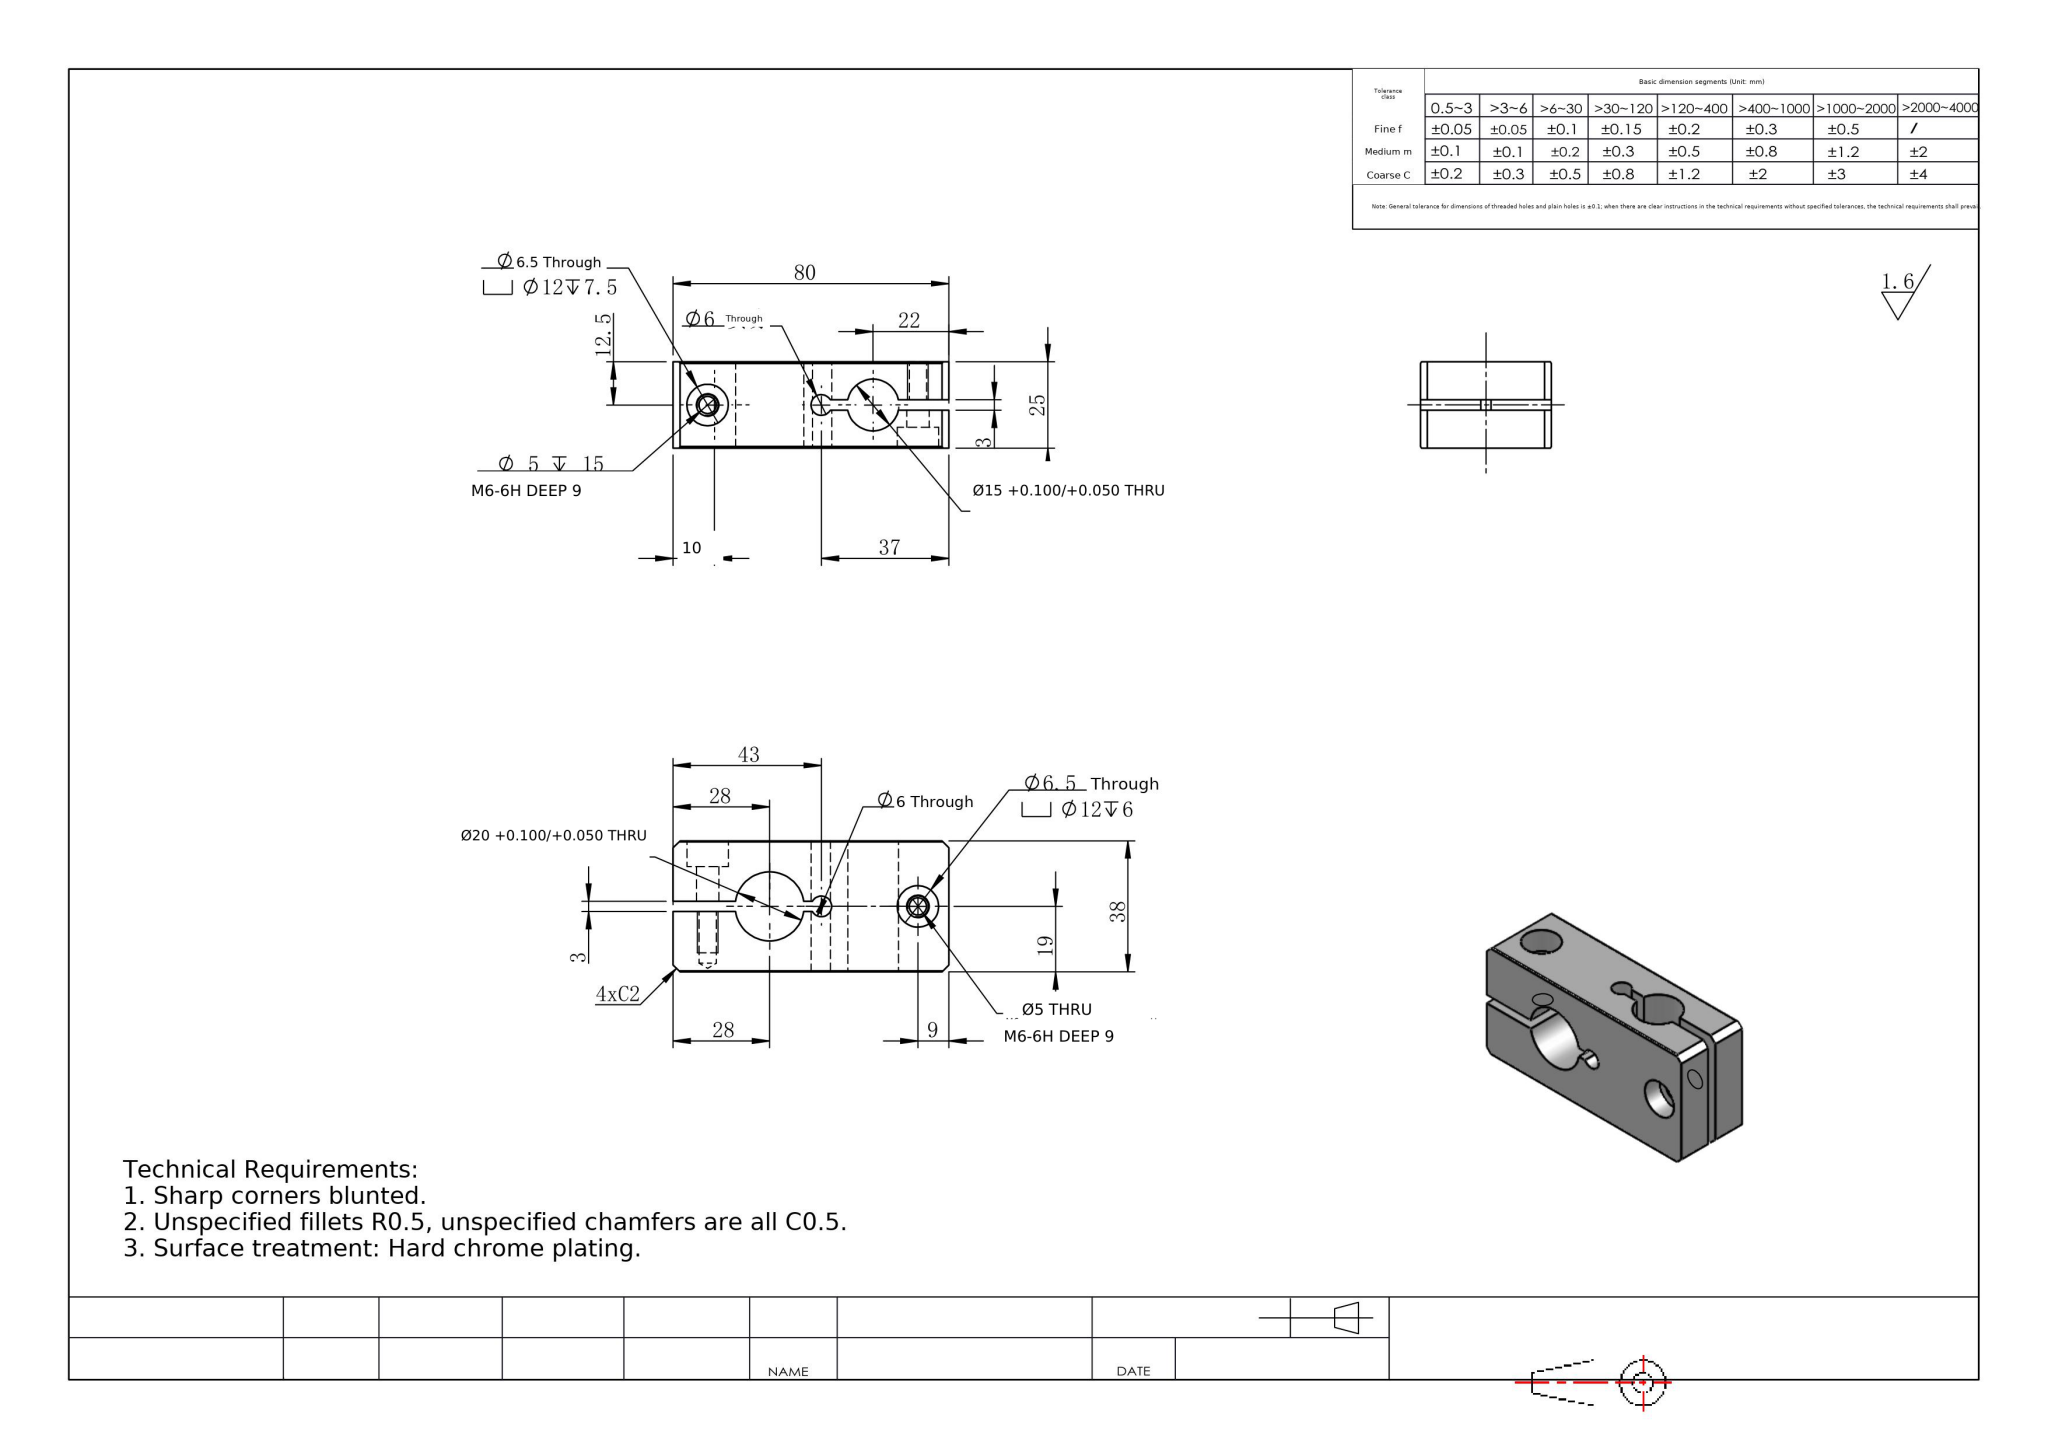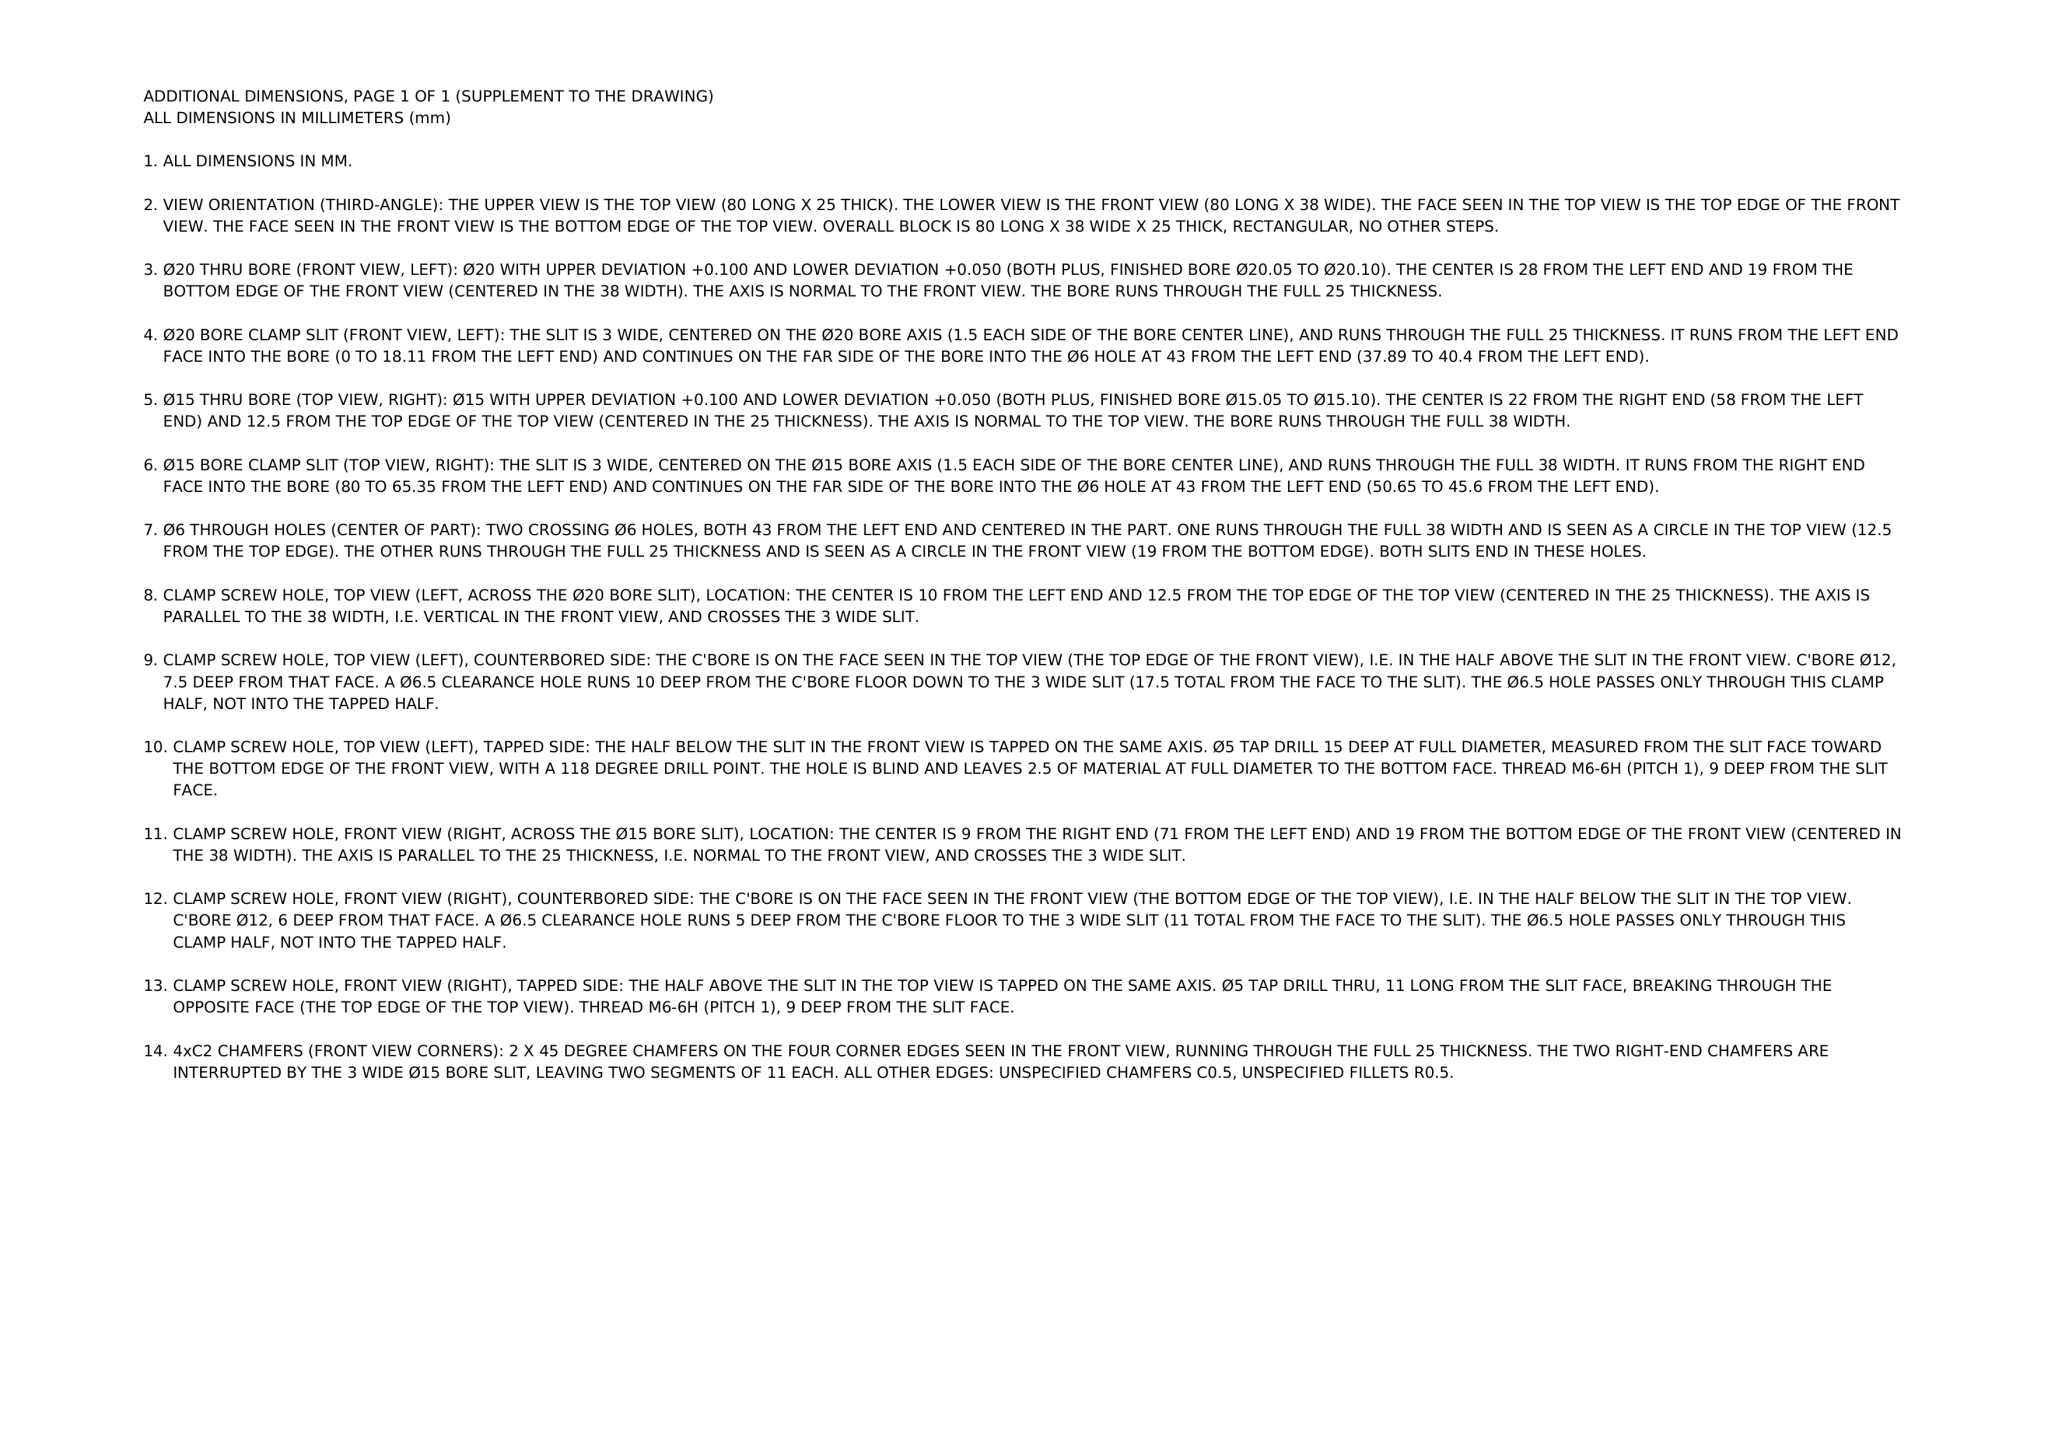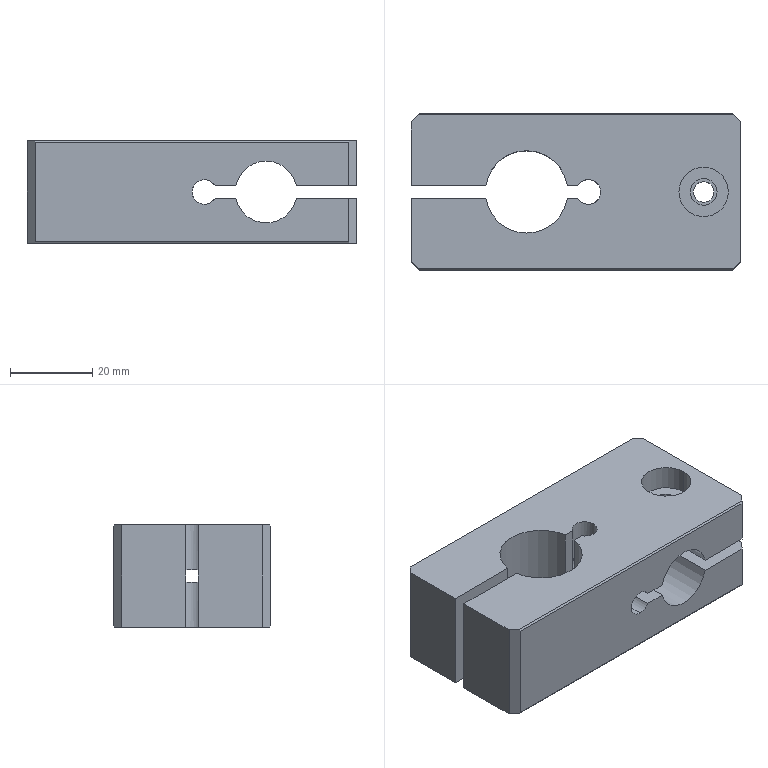Part | NX | mm | 1 solid | 55 faces | box 80 x 38 x 25 mm | volume 53334 mm3 | cylinder 29 | plane 24 | cone 2 | commonest cylinder face diameters 6 x8 6.5 x4 5 x4 12 x4 45 x4 15 x3 20 x2